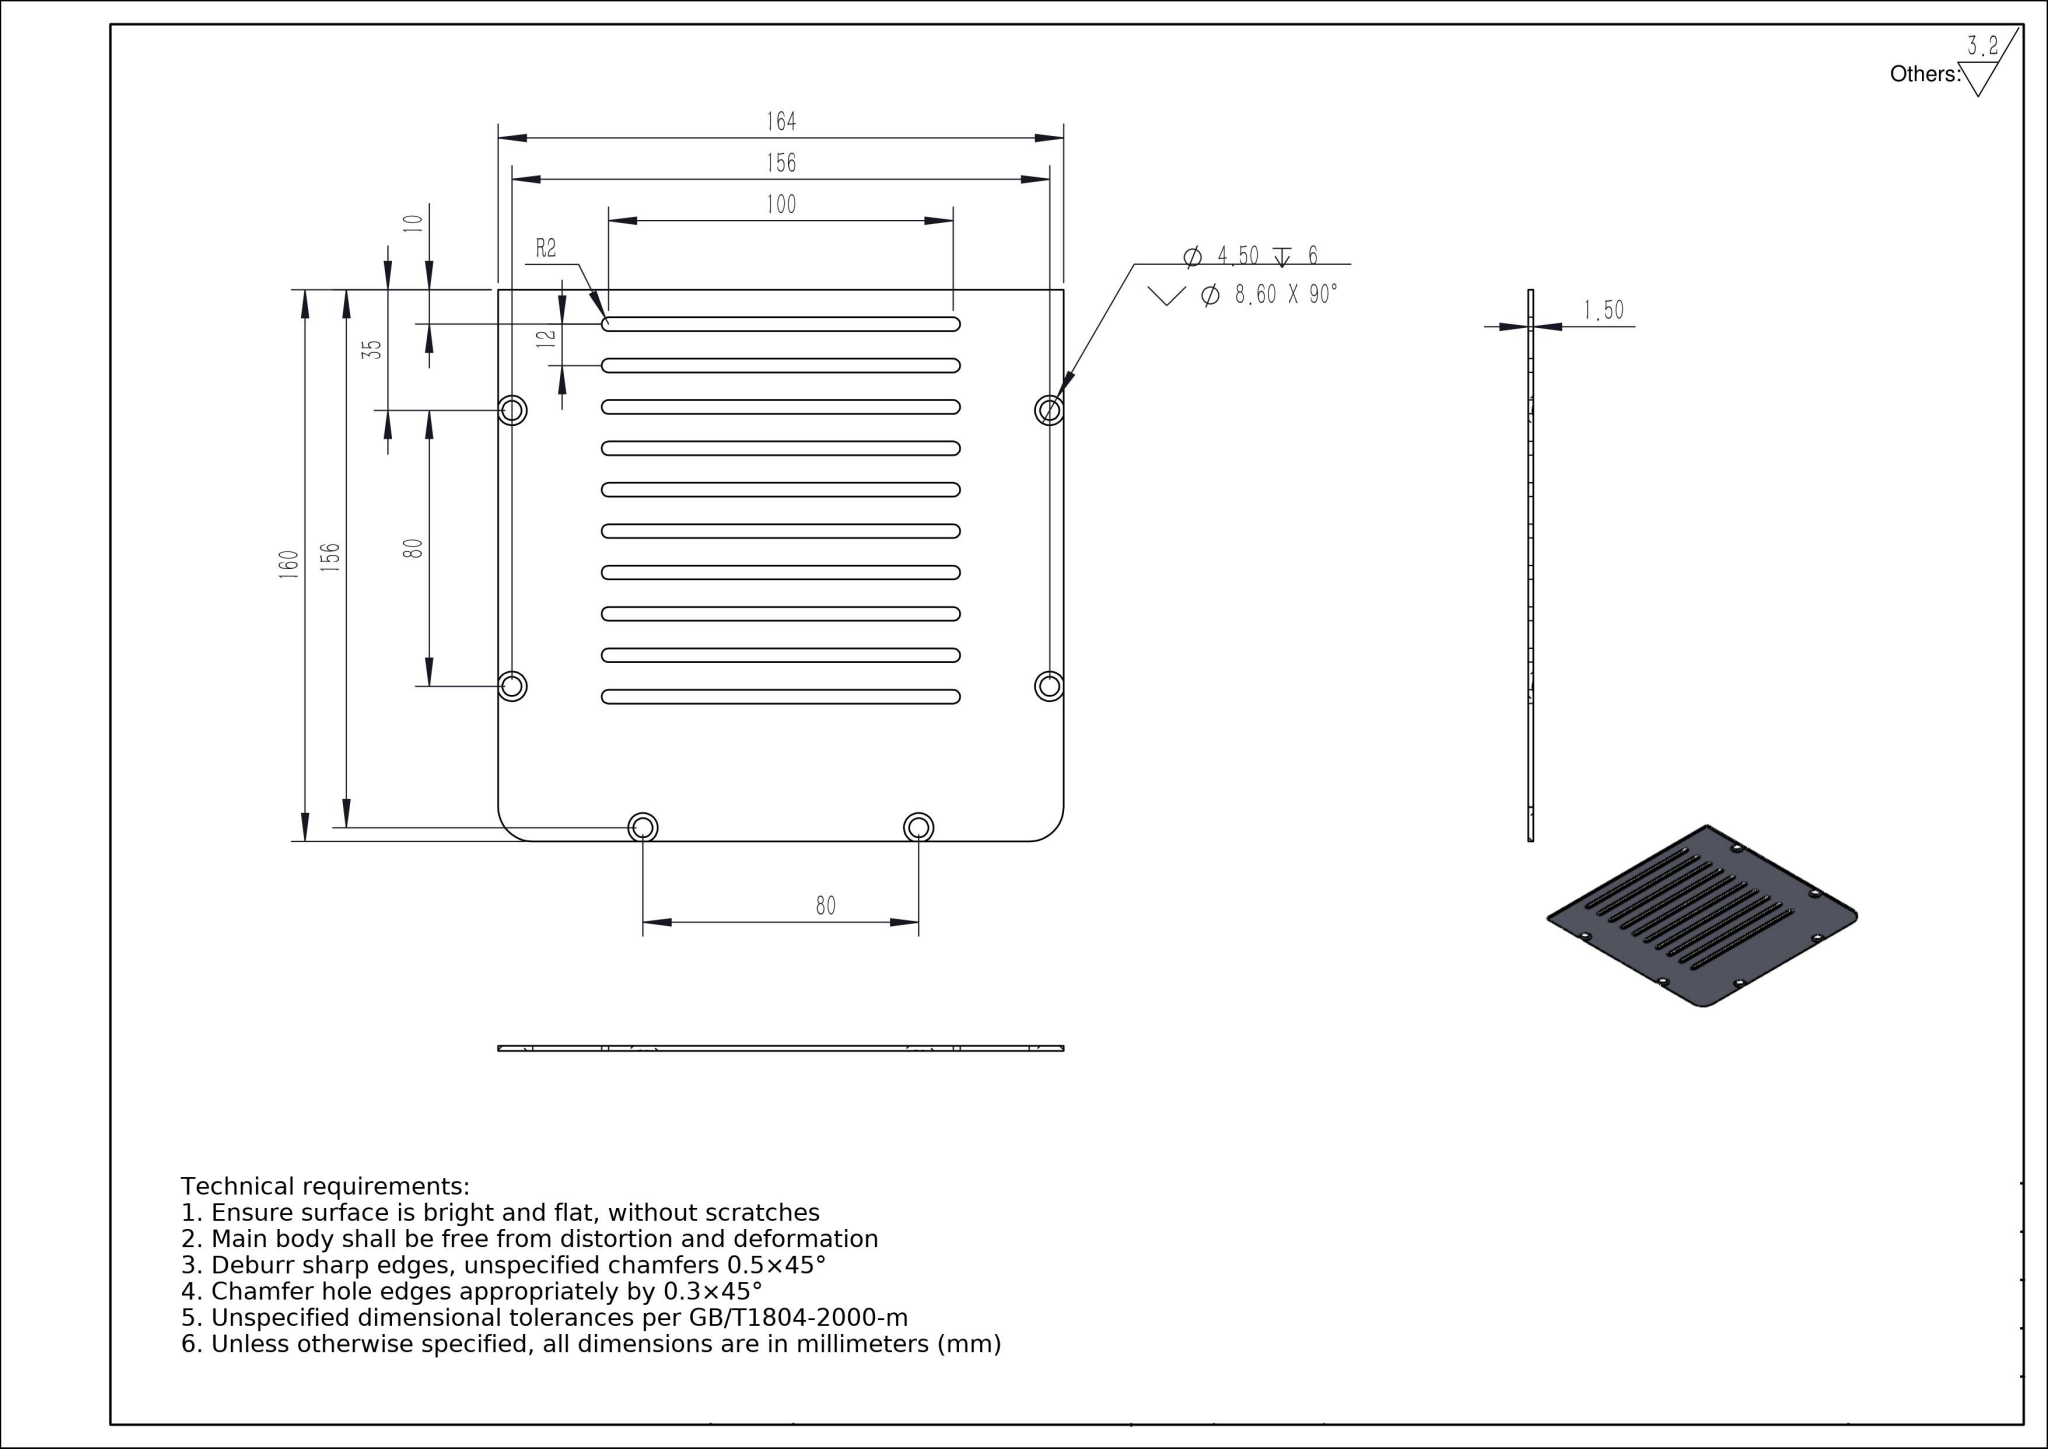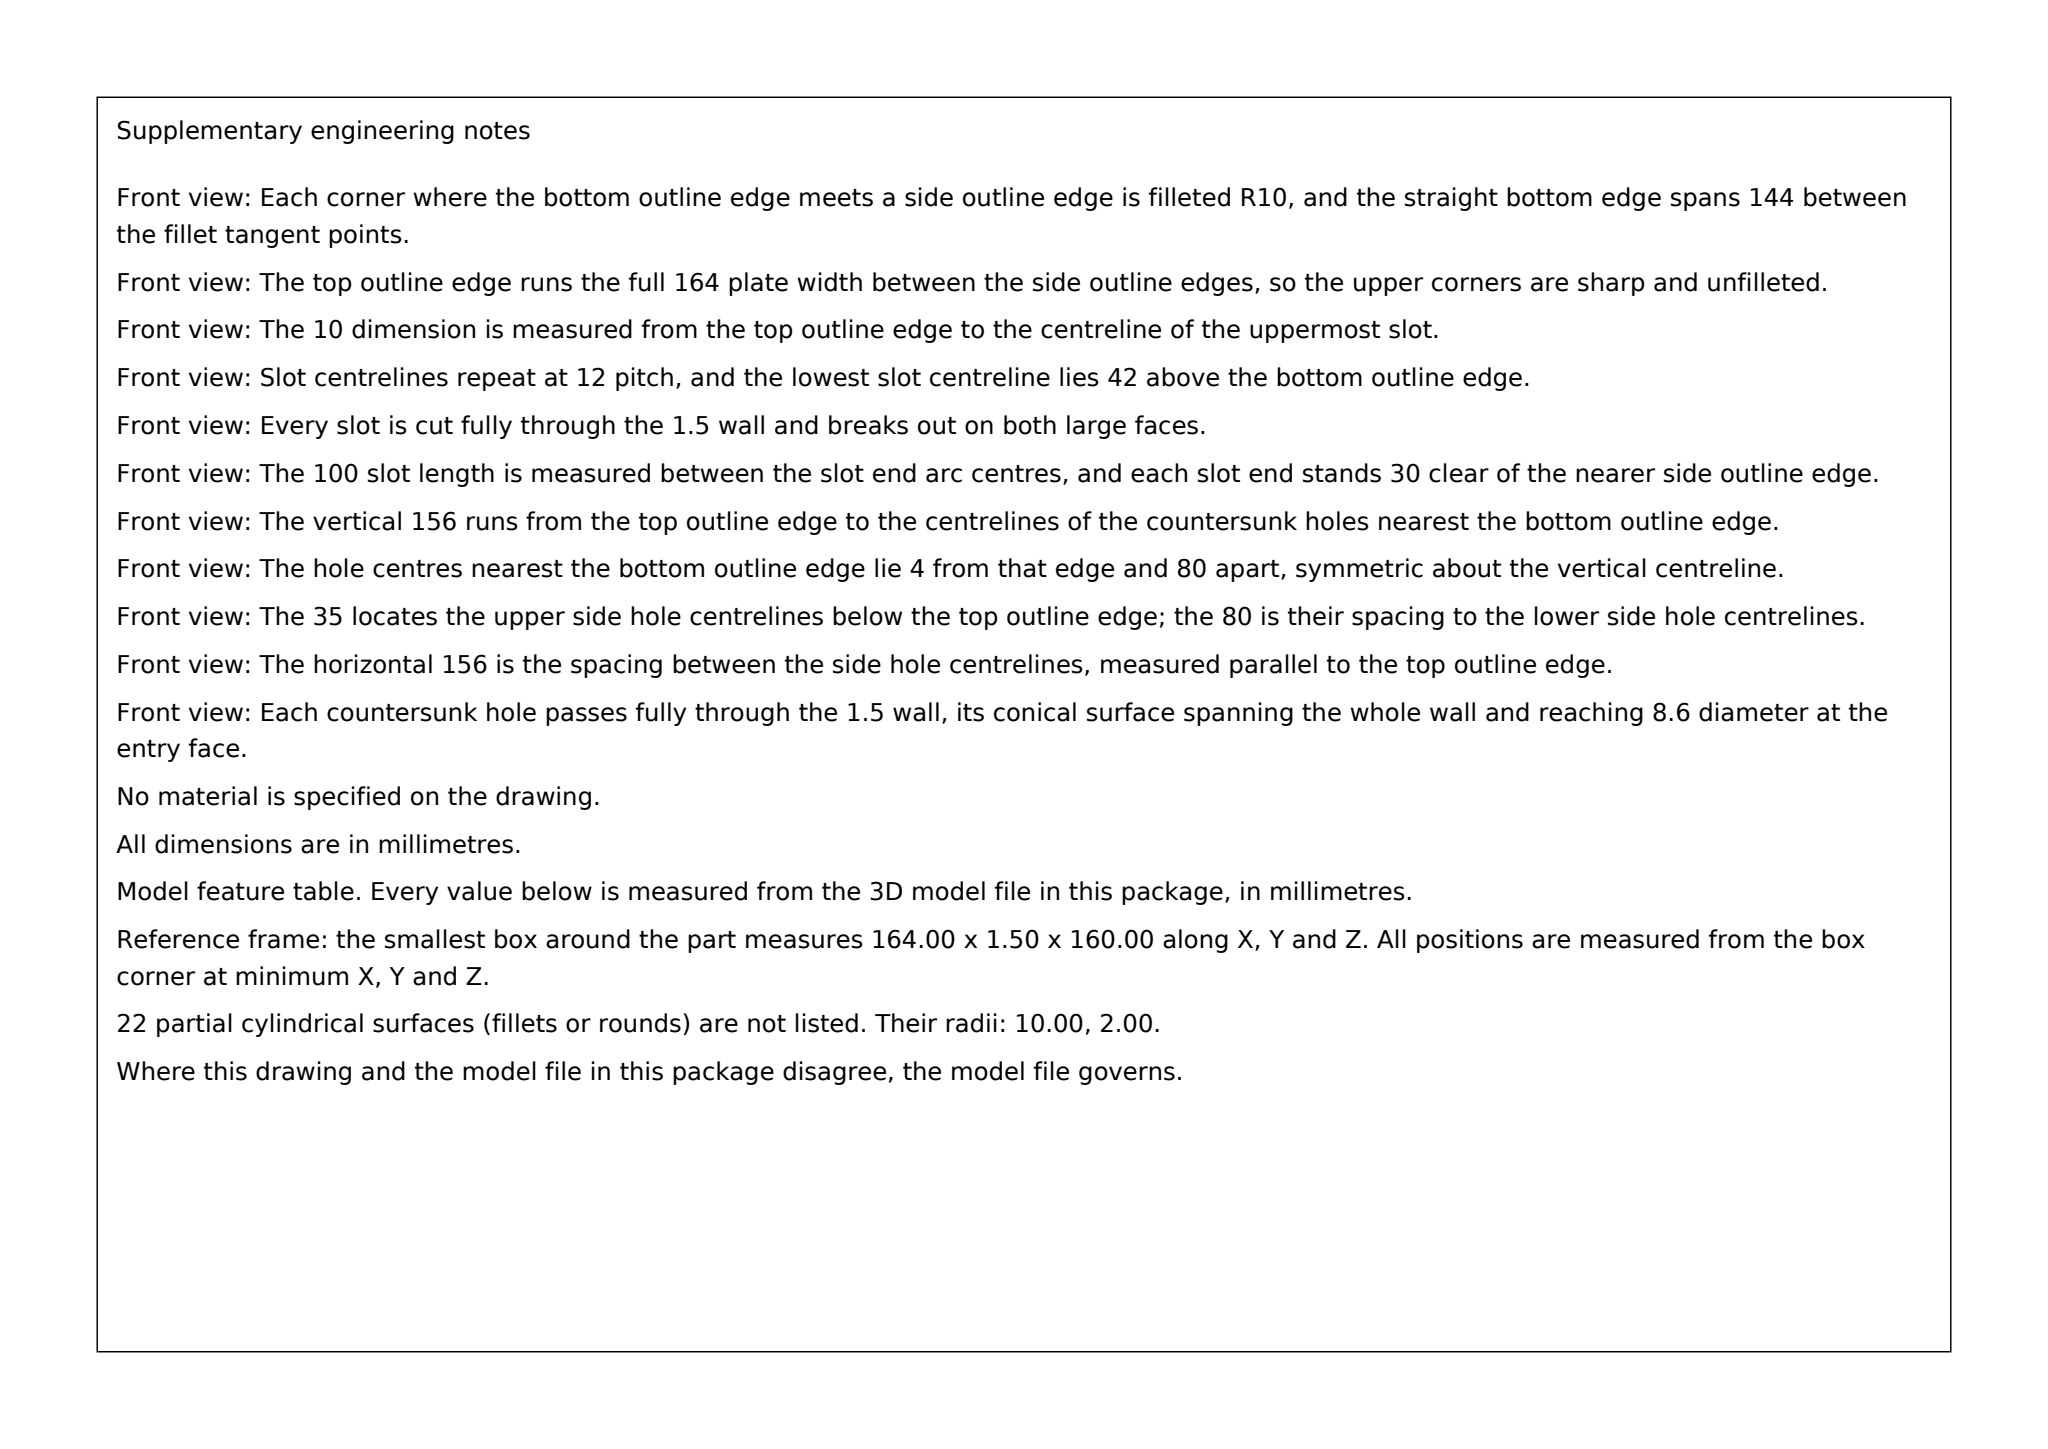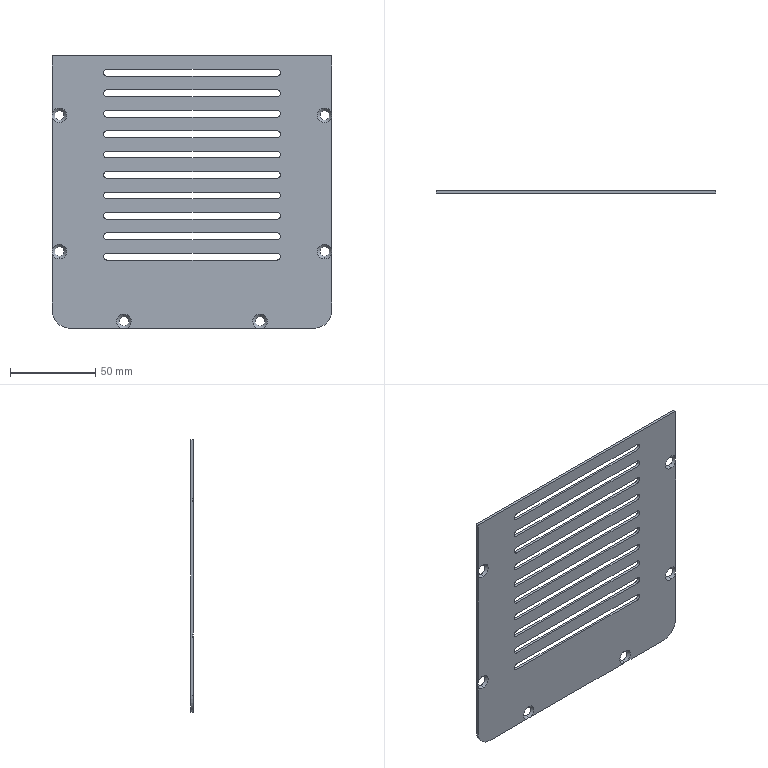Part | SolidWorks | mm | 1 solid | 60 faces | box 164 x 1.5 x 160 mm | volume 32746 mm3 | plane 26 | cylinder 22 | cone 12 | commonest cylinder face diameters 4 x20 20 x2
Drawing notes:
6X MTG HOLE: Ø8.60 X 90° CSK BOTH FACES | from the solid: cones[90.0,8.6] count=12 = 2 cones per hole on 6 holes
MTG HOLE THRU 1.50 PLT; CSKS MEET AT MID-THK, MIN Ø7.10 | from the solid: no cylinder for mtg holes; 1.5 thk plate, 8.6-2x0.75 = 7.10 at mid
6X MTG HOLE; 10X LOUVER SLOT | from the solid: 12 cones/2 = 6 holes; 10 slot pairs of Ø4 cyls at x=32.3 & 132.3
10X SLOT GRP SYM ABOUT PLATE VERT C/L; END C/L 32 FM LH EDGE | from the solid: slot ends x=32.3/132.3 vs plate x=0.3 to 164.3, ctr 82.3
10X SLOT 4 WIDE X 104 OA LG, R2 ENDS, 100 BTWN END C/L | from the solid: Ø4.0 end cyls at x=32.3 and 132.3, 100 apart
2X BTM Ø4.50 HOLES SYM ABOUT VERT CL: 42 FROM EACH SIDE EDGE | from the solid: Part sym about x=82.3 (edges x=0.3/164.3, R10 at x=10.3 & 154.3, slots 30.3-134.3); 80 spacing centered -> holes at x=42.3 & 122.3, i.e. 42 from each edge
L/R Ø4.50 HOLE COLS SYM ABOUT VERT CL OF 164: 4 FROM SIDE EDGE | from the solid: Width 164 (x=0.3 to 164.3), model sym about x=82.3; 156 col spacing centered -> cols at x=4.3 & 160.3 = 4 from each side edge